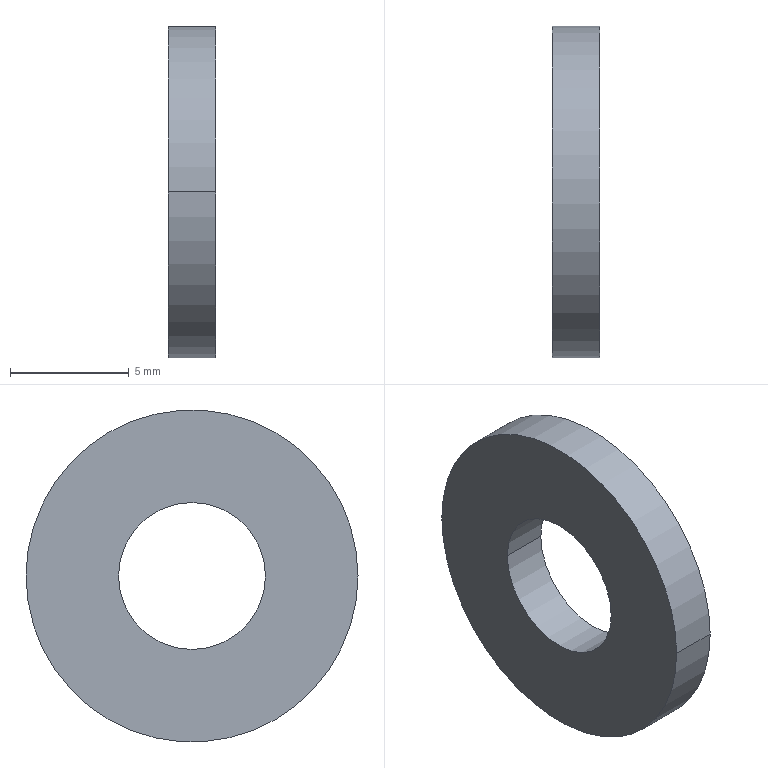Component | SolidWorks | ClampingArm2-1_A78-1 | 1 solid | 6 faces | box 2 x 14 x 14 mm | volume 247 mm3 | cylinder 4 | plane 2 | commonest cylinder face diameters 6.2 x2 14 x2 | material S45C
build123d program:
from build123d import *

# Parameters (mm, degrees)
SKETCH1_R           = 7
SKETCH1_R_2         = 3.1
BOSS_EXTRUDE1_DEPTH = 2


with BuildPart() as part:
    # Sketch1 → Boss-Extrude1 (new body)
    with BuildSketch(Plane(origin=(0, 0, 0), x_dir=(0, 0, -1), z_dir=(1, 0, 0))):
        Circle(SKETCH1_R)
        Circle(SKETCH1_R_2, mode=Mode.SUBTRACT)
    extrude(amount=BOSS_EXTRUDE1_DEPTH)


solid = part.part

# Placed as in the assembly
solid = solid.moved(Location((-14.551, 66.046, -22.5), (0, 0, 0)))
STEP:
#1=CARTESIAN_POINT('',(-0.4941,2.722,-0.8859));
#2=VERTEX_POINT('',#1);
#3=CARTESIAN_POINT('',(-0.4941,2.478,-0.8858));
#4=VERTEX_POINT('',#3);
#5=CARTESIAN_POINT('',(-0.4941,2.6,-0.8858));
#6=DIRECTION('',(1.,0.,0.));
#7=DIRECTION('',(0.,-1.,0.0003333));
#8=AXIS2_PLACEMENT_3D('',#5,#6,#7);
#9=CIRCLE('',#8,0.122);
#10=EDGE_CURVE('',#2,#4,#9,.T.);
#11=ORIENTED_EDGE('',*,*,#10,.T.);
#12=CARTESIAN_POINT('',(-0.5729,2.478,-0.8858));
#13=VERTEX_POINT('',#12);
#14=CARTESIAN_POINT('',(-0.4941,2.478,-0.8858));
#15=DIRECTION('',(-1.,-0.,-0.));
#16=VECTOR('',#15,39.37);
#17=LINE('',#14,#16);
#18=EDGE_CURVE('',#4,#13,#17,.T.);
#19=ORIENTED_EDGE('',*,*,#18,.T.);
#20=CARTESIAN_POINT('',(-0.5729,2.722,-0.8859));
#21=VERTEX_POINT('',#20);
#22=CARTESIAN_POINT('',(-0.5729,2.6,-0.8858));
#23=DIRECTION('',(1.,0.,0.));
#24=DIRECTION('',(0.,-1.,0.0003333));
#25=AXIS2_PLACEMENT_3D('',#22,#23,#24);
#26=CIRCLE('',#25,0.122);
#27=EDGE_CURVE('',#21,#13,#26,.T.);
#28=ORIENTED_EDGE('',*,*,#27,.F.);
#29=CARTESIAN_POINT('',(-0.4941,2.722,-0.8859));
#30=DIRECTION('',(-1.,-0.,-0.));
#31=VECTOR('',#30,39.37);
#32=LINE('',#29,#31);
#33=EDGE_CURVE('',#2,#21,#32,.T.);
#34=ORIENTED_EDGE('',*,*,#33,.F.);
#35=EDGE_LOOP('',(#11,#19,#28,#34));
#36=FACE_OUTER_BOUND('',#35,.T.);
#37=CARTESIAN_POINT('',(-0.4941,2.6,-0.8858));
#38=DIRECTION('',(-1.,-0.,-0.));
#39=DIRECTION('',(0.,1.,-0.0003333));
#40=AXIS2_PLACEMENT_3D('',#37,#38,#39);
#41=CYLINDRICAL_SURFACE('',#40,0.122);
#42=ADVANCED_FACE('',(#36),#41,.F.);
#43=CARTESIAN_POINT('',(-0.4941,2.325,-0.8857));
#44=VERTEX_POINT('',#43);
#45=CARTESIAN_POINT('',(-0.4941,2.876,-0.8859));
#46=VERTEX_POINT('',#45);
#47=CARTESIAN_POINT('',(-0.4941,2.6,-0.8858));
#48=DIRECTION('',(1.,0.,0.));
#49=DIRECTION('',(0.,-1.,0.0003333));
#50=AXIS2_PLACEMENT_3D('',#47,#48,#49);
#51=CIRCLE('',#50,0.2756);
#52=EDGE_CURVE('',#44,#46,#51,.T.);
#53=ORIENTED_EDGE('',*,*,#52,.F.);
#54=CARTESIAN_POINT('',(-0.5729,2.325,-0.8857));
#55=VERTEX_POINT('',#54);
#56=CARTESIAN_POINT('',(-0.4941,2.325,-0.8857));
#57=DIRECTION('',(-1.,-0.,-0.));
#58=VECTOR('',#57,39.37);
#59=LINE('',#56,#58);
#60=EDGE_CURVE('',#44,#55,#59,.T.);
#61=ORIENTED_EDGE('',*,*,#60,.T.);
#62=CARTESIAN_POINT('',(-0.5729,2.876,-0.8859));
#63=VERTEX_POINT('',#62);
#64=CARTESIAN_POINT('',(-0.5729,2.6,-0.8858));
#65=DIRECTION('',(1.,0.,0.));
#66=DIRECTION('',(0.,-1.,0.0003333));
#67=AXIS2_PLACEMENT_3D('',#64,#65,#66);
#68=CIRCLE('',#67,0.2756);
#69=EDGE_CURVE('',#55,#63,#68,.T.);
#70=ORIENTED_EDGE('',*,*,#69,.T.);
#71=CARTESIAN_POINT('',(-0.4941,2.876,-0.8859));
#72=DIRECTION('',(-1.,-0.,-0.));
#73=VECTOR('',#72,39.37);
#74=LINE('',#71,#73);
#75=EDGE_CURVE('',#46,#63,#74,.T.);
#76=ORIENTED_EDGE('',*,*,#75,.F.);
#77=EDGE_LOOP('',(#53,#61,#70,#76));
#78=FACE_OUTER_BOUND('',#77,.T.);
#79=CARTESIAN_POINT('',(-0.4941,2.6,-0.8858));
#80=DIRECTION('',(-1.,-0.,-0.));
#81=DIRECTION('',(0.,1.,-0.0003333));
#82=AXIS2_PLACEMENT_3D('',#79,#80,#81);
#83=CYLINDRICAL_SURFACE('',#82,0.2756);
#84=ADVANCED_FACE('',(#78),#83,.T.);
#85=CARTESIAN_POINT('',(-0.4941,2.6,-0.8858));
#86=DIRECTION('',(1.,0.,0.));
#87=DIRECTION('',(0.,-1.,0.0003333));
#88=AXIS2_PLACEMENT_3D('',#85,#86,#87);
#89=CIRCLE('',#88,0.2756);
#90=EDGE_CURVE('',#46,#44,#89,.T.);
#91=ORIENTED_EDGE('',*,*,#90,.T.);
#92=ORIENTED_EDGE('',*,*,#52,.T.);
#93=EDGE_LOOP('',(#91,#92));
#94=FACE_OUTER_BOUND('',#93,.T.);
#95=ORIENTED_EDGE('',*,*,#10,.F.);
#96=CARTESIAN_POINT('',(-0.4941,2.6,-0.8858));
#97=DIRECTION('',(1.,0.,0.));
#98=DIRECTION('',(0.,-1.,0.0003333));
#99=AXIS2_PLACEMENT_3D('',#96,#97,#98);
#100=CIRCLE('',#99,0.122);
#101=EDGE_CURVE('',#4,#2,#100,.T.);
#102=ORIENTED_EDGE('',*,*,#101,.F.);
#103=EDGE_LOOP('',(#95,#102));
#104=FACE_BOUND('',#103,.T.);
#105=CARTESIAN_POINT('',(-0.4941,2.6,-0.8858));
#106=DIRECTION('',(1.,0.,0.));
#107=DIRECTION('',(0.,-1.,0.0003333));
#108=AXIS2_PLACEMENT_3D('',#105,#106,#107);
#109=PLANE('',#108);
#110=ADVANCED_FACE('',(#94,#104),#109,.T.);
#111=CARTESIAN_POINT('',(-0.5729,2.6,-0.8858));
#112=DIRECTION('',(1.,0.,0.));
#113=DIRECTION('',(0.,-1.,0.0003333));
#114=AXIS2_PLACEMENT_3D('',#111,#112,#113);
#115=CIRCLE('',#114,0.2756);
#116=EDGE_CURVE('',#63,#55,#115,.T.);
#117=ORIENTED_EDGE('',*,*,#116,.F.);
#118=ORIENTED_EDGE('',*,*,#69,.F.);
#119=EDGE_LOOP('',(#117,#118));
#120=FACE_OUTER_BOUND('',#119,.T.);
#121=ORIENTED_EDGE('',*,*,#27,.T.);
#122=CARTESIAN_POINT('',(-0.5729,2.6,-0.8858));
#123=DIRECTION('',(1.,0.,0.));
#124=DIRECTION('',(0.,-1.,0.0003333));
#125=AXIS2_PLACEMENT_3D('',#122,#123,#124);
#126=CIRCLE('',#125,0.122);
#127=EDGE_CURVE('',#13,#21,#126,.T.);
#128=ORIENTED_EDGE('',*,*,#127,.T.);
#129=EDGE_LOOP('',(#121,#128));
#130=FACE_BOUND('',#129,.T.);
#131=CARTESIAN_POINT('',(-0.5729,2.6,-0.8858));
#132=DIRECTION('',(1.,0.,0.));
#133=DIRECTION('',(0.,-1.,0.0003333));
#134=AXIS2_PLACEMENT_3D('',#131,#132,#133);
#135=PLANE('',#134);
#136=ADVANCED_FACE('',(#120,#130),#135,.F.);
#137=ORIENTED_EDGE('',*,*,#60,.F.);
#138=ORIENTED_EDGE('',*,*,#90,.F.);
#139=ORIENTED_EDGE('',*,*,#75,.T.);
#140=ORIENTED_EDGE('',*,*,#116,.T.);
#141=EDGE_LOOP('',(#137,#138,#139,#140));
#142=FACE_OUTER_BOUND('',#141,.T.);
#143=CARTESIAN_POINT('',(-0.4941,2.6,-0.8858));
#144=DIRECTION('',(-1.,-0.,-0.));
#145=DIRECTION('',(0.,1.,-0.0003333));
#146=AXIS2_PLACEMENT_3D('',#143,#144,#145);
#147=CYLINDRICAL_SURFACE('',#146,0.2756);
#148=ADVANCED_FACE('',(#142),#147,.T.);
#149=ORIENTED_EDGE('',*,*,#18,.F.);
#150=ORIENTED_EDGE('',*,*,#101,.T.);
#151=ORIENTED_EDGE('',*,*,#33,.T.);
#152=ORIENTED_EDGE('',*,*,#127,.F.);
#153=EDGE_LOOP('',(#149,#150,#151,#152));
#154=FACE_OUTER_BOUND('',#153,.T.);
#155=CARTESIAN_POINT('',(-0.4941,2.6,-0.8858));
#156=DIRECTION('',(-1.,-0.,-0.));
#157=DIRECTION('',(0.,1.,-0.0003333));
#158=AXIS2_PLACEMENT_3D('',#155,#156,#157);
#159=CYLINDRICAL_SURFACE('',#158,0.122);
#160=ADVANCED_FACE('',(#154),#159,.F.);
#161=CLOSED_SHELL('',(#42,#84,#110,#136,#148,#160));
#162=MANIFOLD_SOLID_BREP('',#161);
#163=CARTESIAN_POINT('',(0.,0.,0.));
#164=DIRECTION('',(0.,0.,1.));
#165=DIRECTION('',(1.,0.,0.));
#166=AXIS2_PLACEMENT_3D('',#163,#164,#165);
#167=(LENGTH_UNIT()NAMED_UNIT(*)SI_UNIT($,.METRE.));
#168=LENGTH_MEASURE_WITH_UNIT(LENGTH_MEASURE(0.0254),#167);
#169=DIMENSIONAL_EXPONENTS(1.,0.,0.,0.,0.,0.,0.);
#170=(CONVERSION_BASED_UNIT('',#168)LENGTH_UNIT()NAMED_UNIT(#169));
#171=UNCERTAINTY_MEASURE_WITH_UNIT(LENGTH_MEASURE(0.00001),#170,'','');
#172=(NAMED_UNIT(*)PLANE_ANGLE_UNIT()SI_UNIT($,.RADIAN.));
#173=(NAMED_UNIT(*)SI_UNIT($,.STERADIAN.)SOLID_ANGLE_UNIT());
#174=(GEOMETRIC_REPRESENTATION_CONTEXT(3)GLOBAL_UNCERTAINTY_ASSIGNED_CONTEXT((#171))GLOBAL_UNIT_ASSIGNED_CONTEXT((#170,#172,#173))REPRESENTATION_CONTEXT('',''));
#175=ADVANCED_BREP_SHAPE_REPRESENTATION('',(#162,#166),#174);
#176=COLOUR_RGB('',0.7922,0.8196,0.9333);
#177=FILL_AREA_STYLE_COLOUR('',#176);
#178=FILL_AREA_STYLE('',(#177));
#179=SURFACE_STYLE_FILL_AREA(#178);
#180=SURFACE_SIDE_STYLE('',(#179));
#181=SURFACE_STYLE_USAGE(.BOTH.,#180);
#182=PRESENTATION_STYLE_ASSIGNMENT((#181));
#183=STYLED_ITEM('',(#182),#162);
#184=PRESENTATION_LAYER_ASSIGNMENT('','',(#183));
#185=(LENGTH_UNIT()NAMED_UNIT(*)SI_UNIT($,.METRE.));
#186=LENGTH_MEASURE_WITH_UNIT(LENGTH_MEASURE(0.0254),#185);
#187=DIMENSIONAL_EXPONENTS(1.,0.,0.,0.,0.,0.,0.);
#188=(CONVERSION_BASED_UNIT('',#186)LENGTH_UNIT()NAMED_UNIT(#187));
#189=UNCERTAINTY_MEASURE_WITH_UNIT(LENGTH_MEASURE(0.00001),#188,'','');
#190=(NAMED_UNIT(*)PLANE_ANGLE_UNIT()SI_UNIT($,.RADIAN.));
#191=(NAMED_UNIT(*)SI_UNIT($,.STERADIAN.)SOLID_ANGLE_UNIT());
#192=(GEOMETRIC_REPRESENTATION_CONTEXT(3)GLOBAL_UNCERTAINTY_ASSIGNED_CONTEXT((#189))GLOBAL_UNIT_ASSIGNED_CONTEXT((#188,#190,#191))REPRESENTATION_CONTEXT('',''));
#193=MECHANICAL_DESIGN_GEOMETRIC_PRESENTATION_REPRESENTATION('',(#183),#192);